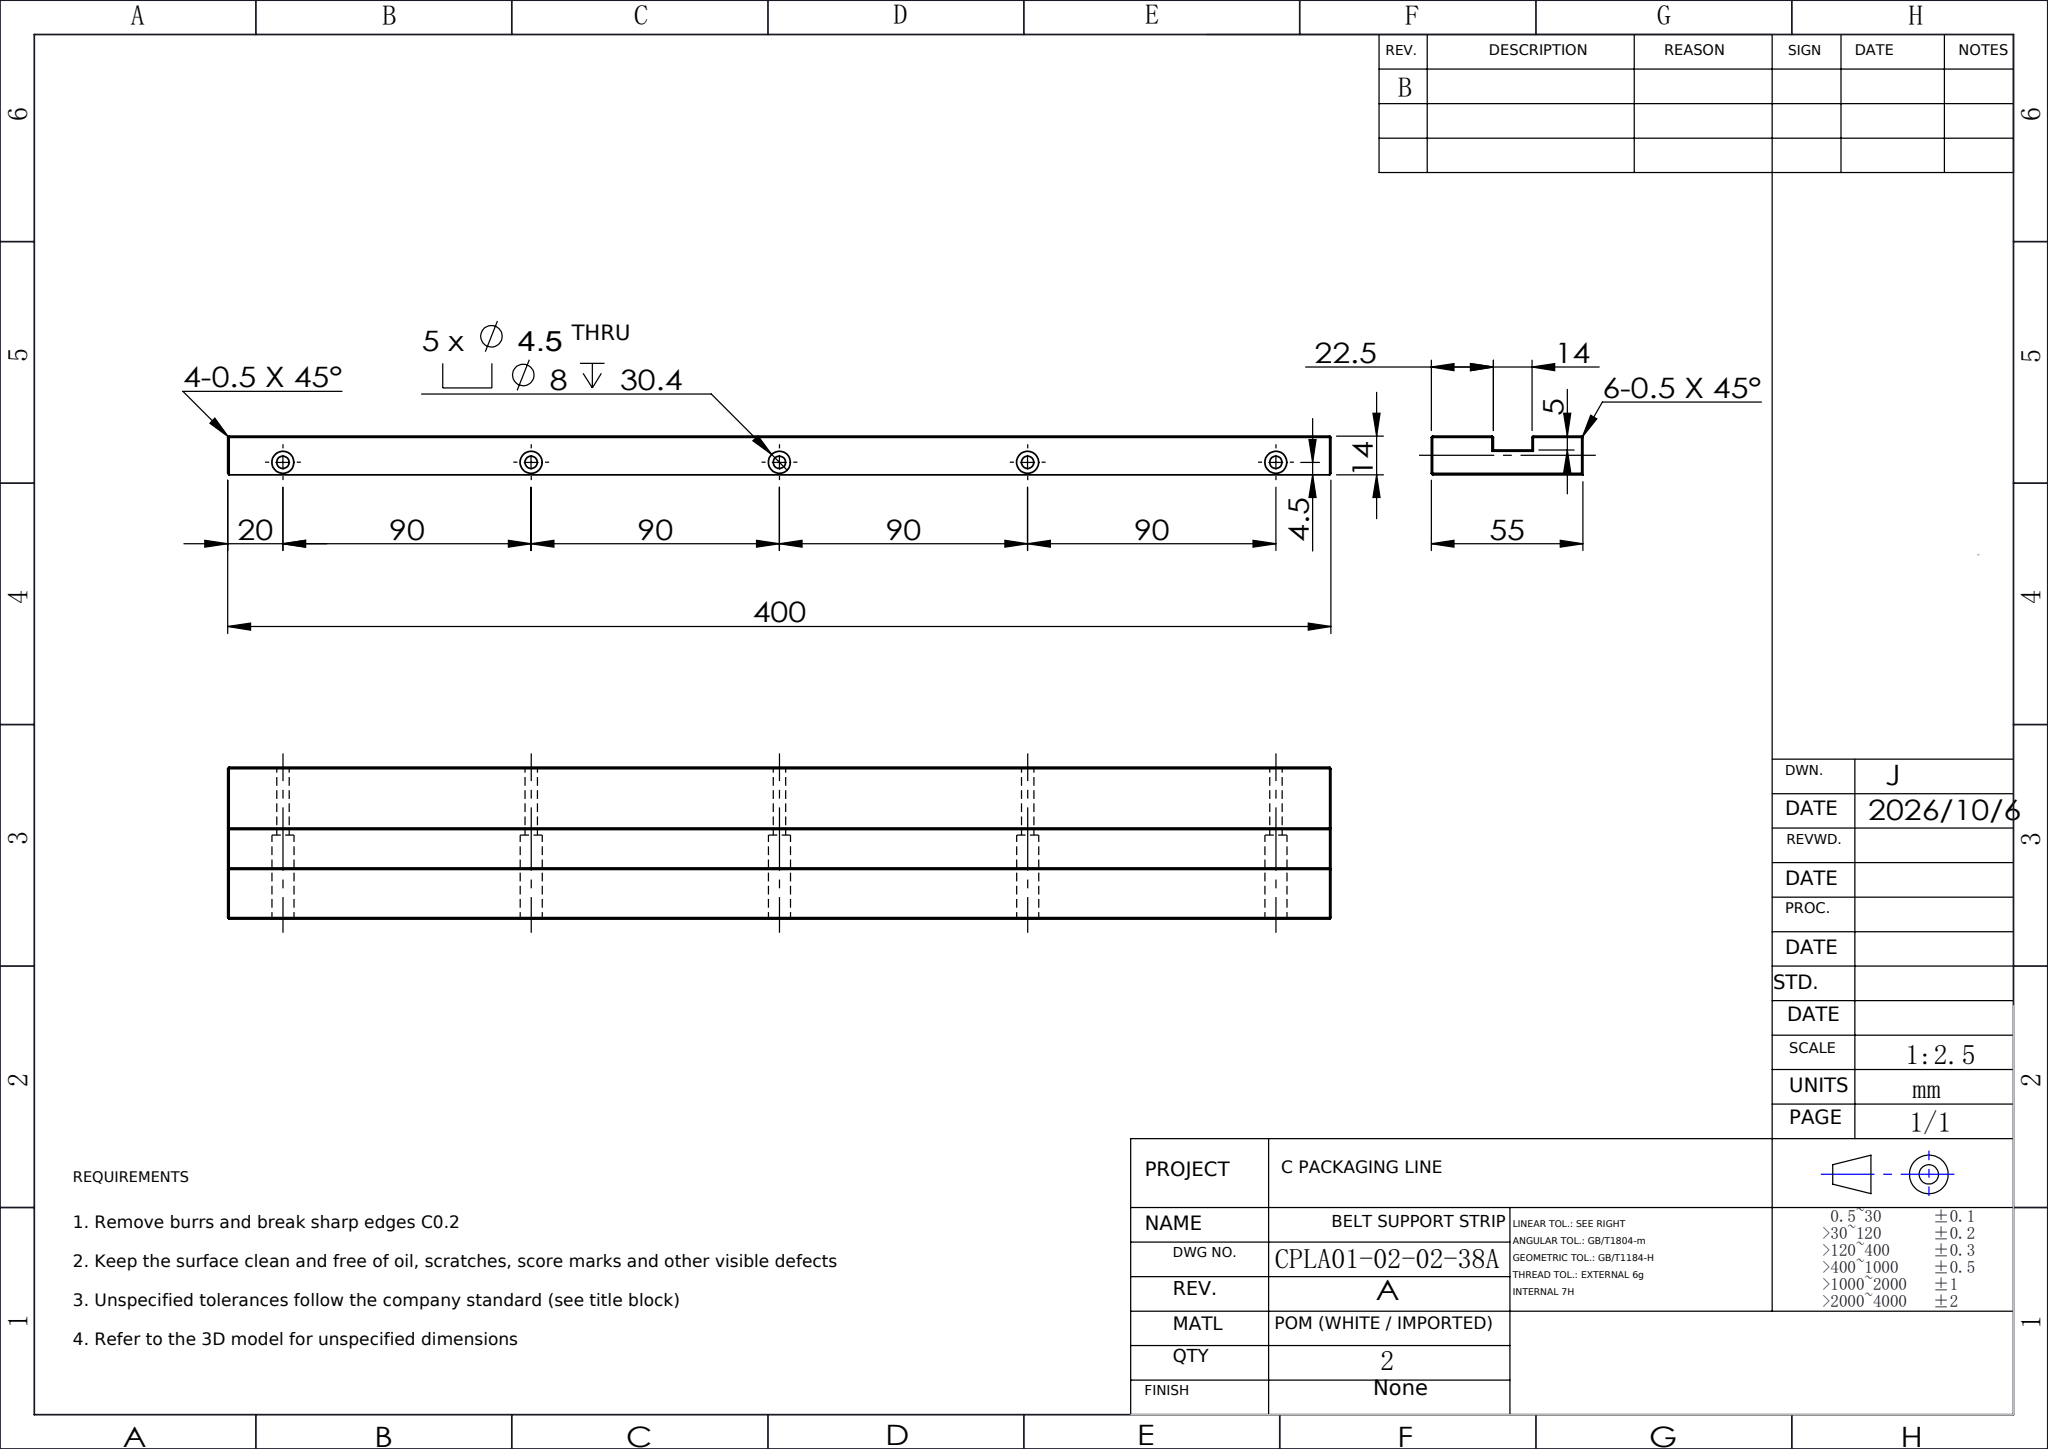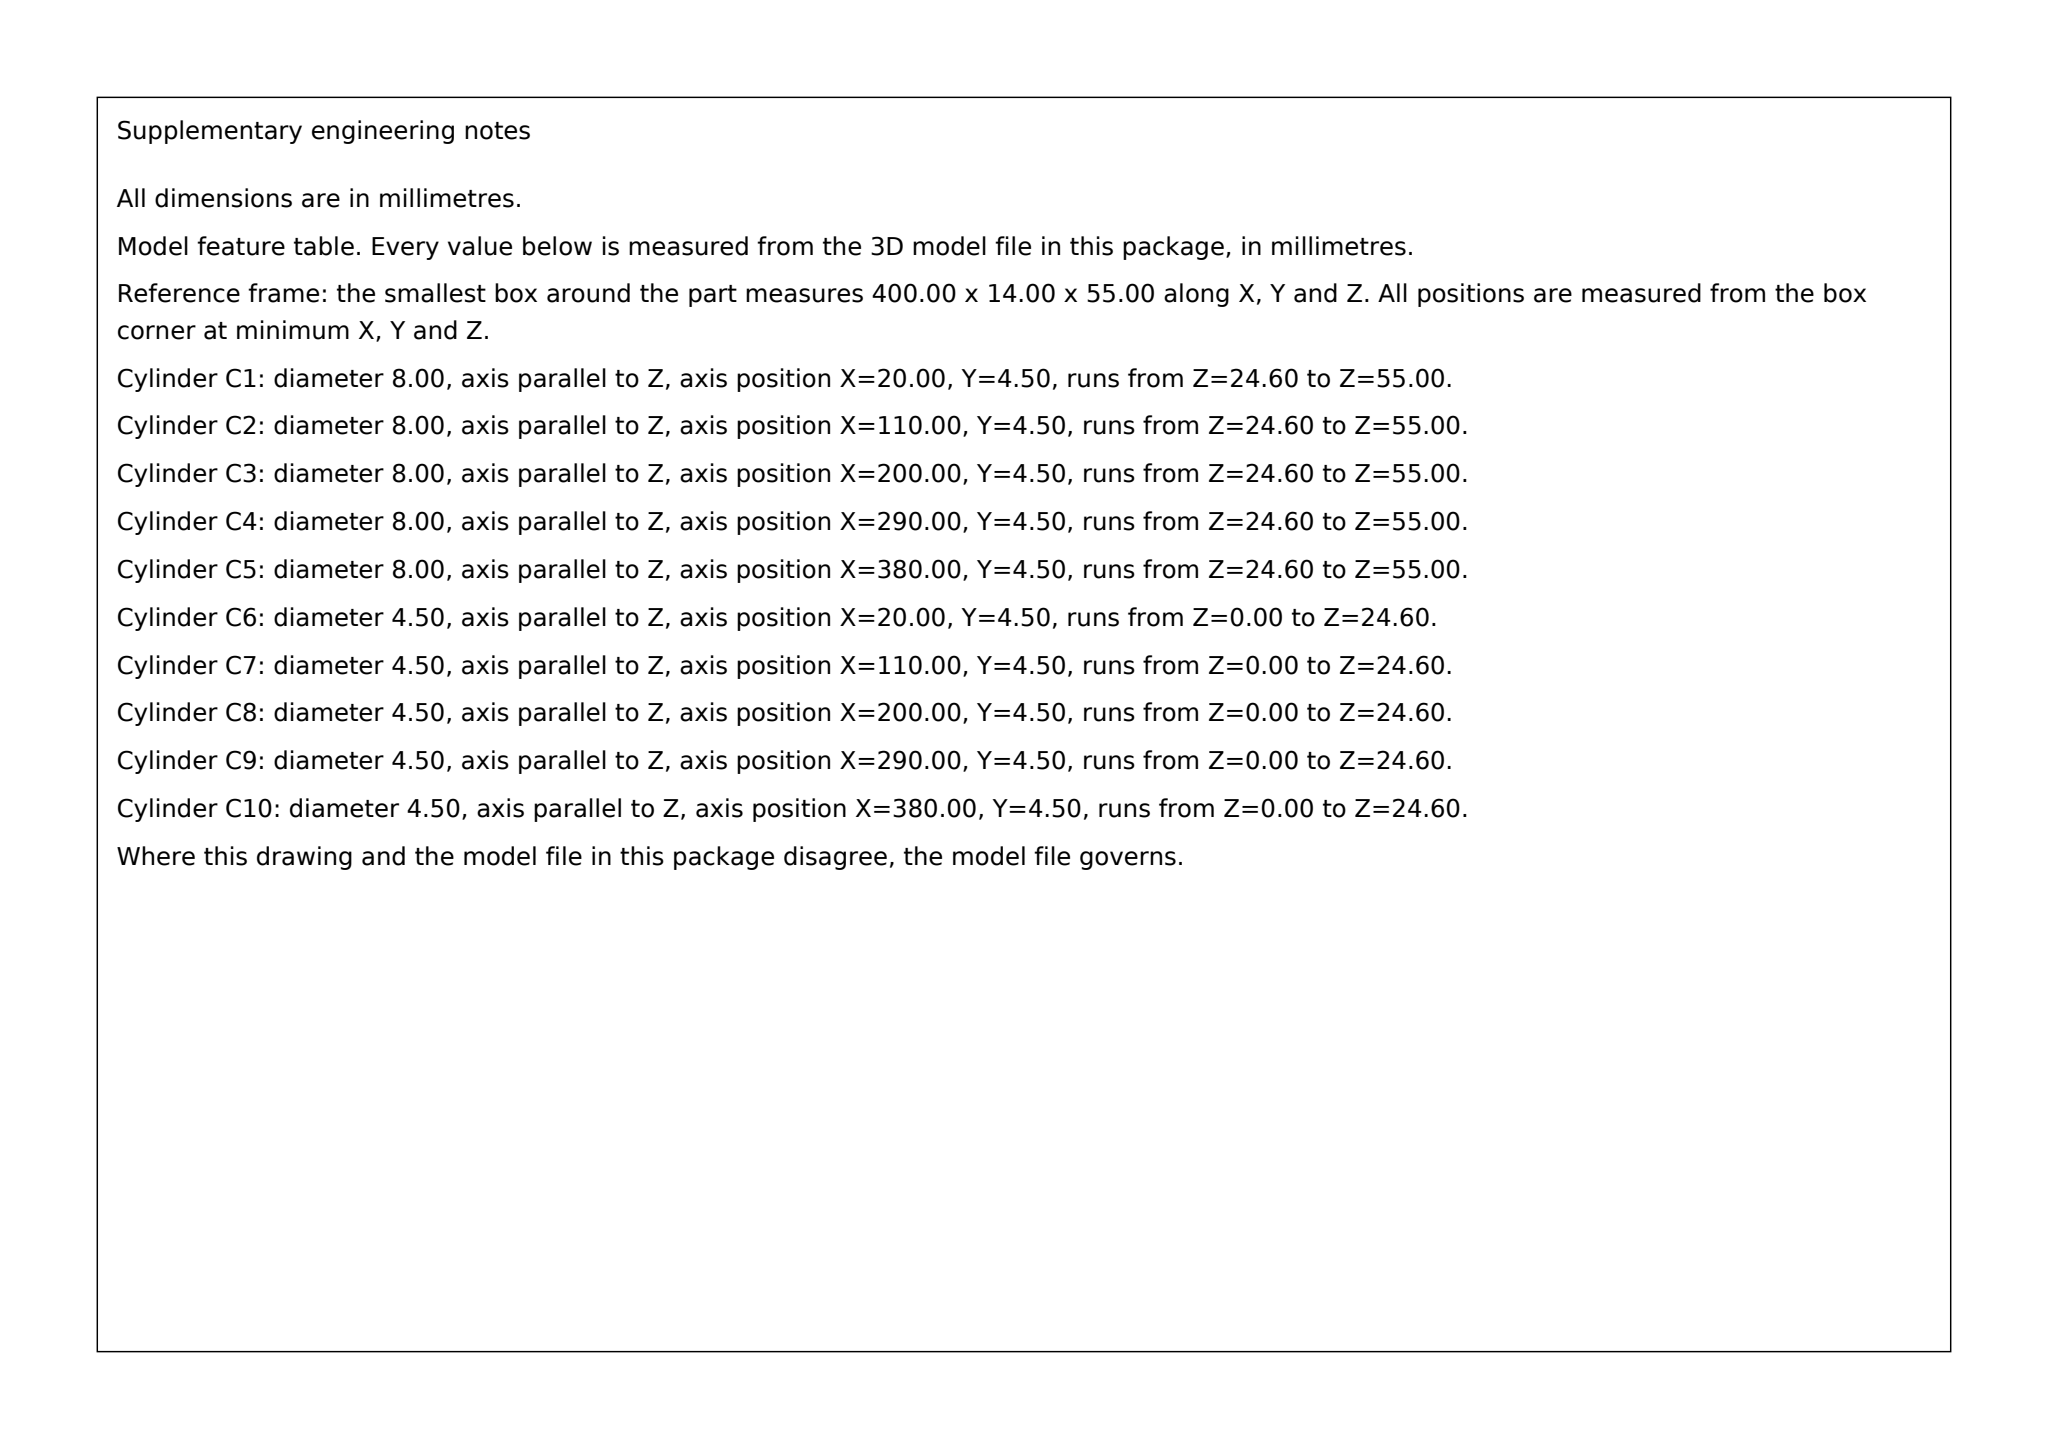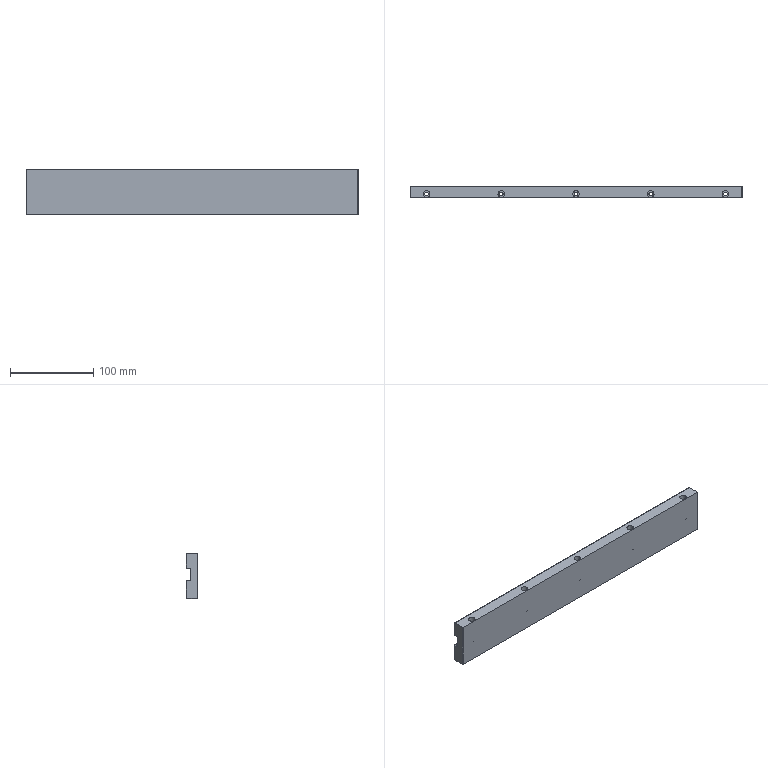Part | SolidWorks | mm | 1 solid | 66 faces | box 400 x 14 x 55 mm | volume 270117 mm3 | plane 46 | cylinder 20 | commonest cylinder face diameters 8 x10 4.5 x10
build123d program:
from build123d import *

# Parameters (mm, degrees)
SKETCH1_W                                       = 400
SKETCH1_H                                       = 14
BOSS_EXTRUDE1_DEPTH                             = 27.5
CUT_EXTRUDE1_START                              = -2
SKETCH6_W                                       = 400
SKETCH6_H                                       = 5
CUT_EXTRUDE1_DEPTH                              = 7
M4_HEX_SOCKET_HEAD_CAP_SCREW_CBORE1_D           = 4.5
M4_HEX_SOCKET_HEAD_CAP_SCREW_CBORE1_CBORE_D     = 8
M4_HEX_SOCKET_HEAD_CAP_SCREW_CBORE1_CBORE_DEPTH = 30.4
CHAMFER1_SIZE                                   = 0.5


with BuildPart() as part:
    # Sketch1 → Boss-Extrude1 (new, symmetric)
    with BuildSketch(Plane.XY):
        Rectangle(SKETCH1_W, SKETCH1_H)
    extrude(amount=BOSS_EXTRUDE1_DEPTH, both=True)

    # Sketch6 → Cut-Extrude1 (cut, symmetric)
    with BuildSketch(Plane(origin=(0, 0, 0), x_dir=(-1, 0, 0), z_dir=(0, 0, -1)).offset(CUT_EXTRUDE1_START)):
        with Locations((0, 4.5)):
            Rectangle(SKETCH6_W, SKETCH6_H)
    extrude(amount=CUT_EXTRUDE1_DEPTH, both=True, mode=Mode.SUBTRACT)

    # M4 Hex Socket Head Cap Screw CBORE1 (through all)
    with Locations(Plane.XY.offset(27.5)):
        with Locations((-90, -2.5), (90, -2.5), (0, -2.5), (-180, -2.5), (180, -2.5)):
            CounterBoreHole(M4_HEX_SOCKET_HEAD_CAP_SCREW_CBORE1_D / 2, M4_HEX_SOCKET_HEAD_CAP_SCREW_CBORE1_CBORE_D / 2, M4_HEX_SOCKET_HEAD_CAP_SCREW_CBORE1_CBORE_DEPTH)

    # Chamfer1
    chamfer1_edges = [part.edges().sort_by_distance(p)[0] for p in [
        (-200, 0, 27.5),
        (-200, 7, -16.25),
        (200, 7, -16.25),
        (200, 4.5, 9),
        (200, 2, 2),
        (0, 7, 9),
        (-200, 4.5, 9),
        (-200, 2, 2),
        (200, 4.5, -5),
        (-200, 4.5, -5),
        (0, 7, -5),
        (200, 0, 27.5),
        (0, -7, -27.5),
        (-200, 0, -27.5),
        (0, 7, -27.5),
        (200, 0, -27.5),
        (0, 7, 27.5),
        (200, -7, 0),
        (-200, -7, 0),
        (-200, 7, 18.25),
        (200, 7, 18.25),
    ]]
    chamfer(chamfer1_edges, length=CHAMFER1_SIZE)


solid = part.part